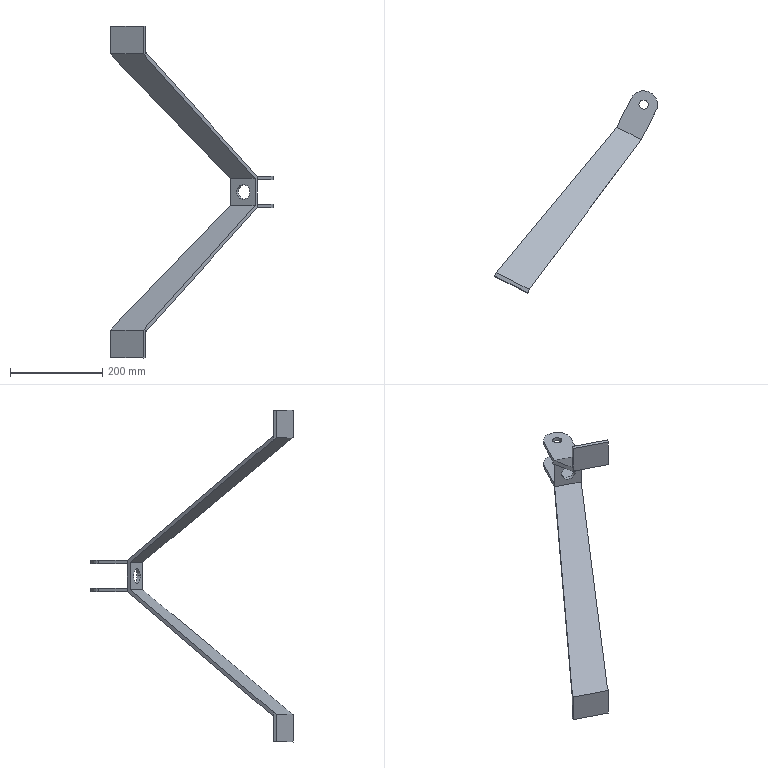Component | SolidWorks | TriangularHanger-1 | 1 solid | 36 faces | box 353.14 x 438.28 x 720 mm | volume 725422 mm3 | plane 26 | cylinder 10 | commonest cylinder face diameters 20 x4 60 x4 32 x2
STEP:
#1=COLOUR_RGB('',0.7922,0.8196,0.9333);
#2=FILL_AREA_STYLE_COLOUR('',#1);
#3=FILL_AREA_STYLE('',(#2));
#4=SURFACE_STYLE_FILL_AREA(#3);
#5=SURFACE_SIDE_STYLE('',(#4));
#6=SURFACE_STYLE_USAGE(.BOTH.,#5);
#7=PRESENTATION_STYLE_ASSIGNMENT((#6));
#8=CARTESIAN_POINT('',(20.97,-29.022,71.377));
#9=VERTEX_POINT('',#8);
#10=CARTESIAN_POINT('',(22.094,-29.591,71.377));
#11=VERTEX_POINT('',#10);
#12=CARTESIAN_POINT('',(21.532,-29.306,71.377));
#13=DIRECTION('',(-0.4521,-0.892,-0.));
#14=DIRECTION('',(0.892,-0.4521,-0.));
#15=AXIS2_PLACEMENT_3D('',#12,#13,#14);
#16=CIRCLE('',#15,0.6299);
#17=EDGE_CURVE('',#9,#11,#16,.T.);
#18=ORIENTED_EDGE('',*,*,#17,.T.);
#19=CARTESIAN_POINT('',(22.236,-29.31,71.377));
#20=VERTEX_POINT('',#19);
#21=CARTESIAN_POINT('',(22.058,-29.661,71.377));
#22=DIRECTION('',(0.4521,0.892,0.));
#23=VECTOR('',#22,39.37);
#24=LINE('',#21,#23);
#25=EDGE_CURVE('',#11,#20,#24,.T.);
#26=ORIENTED_EDGE('',*,*,#25,.T.);
#27=CARTESIAN_POINT('',(21.112,-28.741,71.377));
#28=VERTEX_POINT('',#27);
#29=CARTESIAN_POINT('',(21.674,-29.026,71.377));
#30=DIRECTION('',(0.4521,0.892,0.));
#31=DIRECTION('',(-0.892,0.4521,0.));
#32=AXIS2_PLACEMENT_3D('',#29,#30,#31);
#33=CIRCLE('',#32,0.6299);
#34=EDGE_CURVE('',#20,#28,#33,.T.);
#35=ORIENTED_EDGE('',*,*,#34,.T.);
#36=CARTESIAN_POINT('',(20.934,-29.092,71.377));
#37=DIRECTION('',(0.4521,0.892,0.));
#38=VECTOR('',#37,39.37);
#39=LINE('',#36,#38);
#40=EDGE_CURVE('',#9,#28,#39,.T.);
#41=ORIENTED_EDGE('',*,*,#40,.F.);
#42=EDGE_LOOP('',(#18,#26,#35,#41));
#43=FACE_OUTER_BOUND('',#42,.T.);
#44=CARTESIAN_POINT('',(21.496,-29.377,71.377));
#45=DIRECTION('',(0.4521,0.892,0.));
#46=DIRECTION('',(-0.892,0.4521,0.));
#47=AXIS2_PLACEMENT_3D('',#44,#45,#46);
#48=CYLINDRICAL_SURFACE('',#47,0.6299);
#49=ADVANCED_FACE('',(#43),#48,.F.);
#50=CARTESIAN_POINT('',(22.569,-26.389,70.028));
#51=VERTEX_POINT('',#50);
#52=CARTESIAN_POINT('',(23.271,-26.745,70.028));
#53=VERTEX_POINT('',#52);
#54=CARTESIAN_POINT('',(22.92,-26.567,70.028));
#55=DIRECTION('',(-0.,-0.,1.));
#56=DIRECTION('',(0.892,-0.4521,-0.));
#57=AXIS2_PLACEMENT_3D('',#54,#55,#56);
#58=CIRCLE('',#57,0.3937);
#59=EDGE_CURVE('',#51,#53,#58,.T.);
#60=ORIENTED_EDGE('',*,*,#59,.F.);
#61=CARTESIAN_POINT('',(22.569,-26.389,70.343));
#62=VERTEX_POINT('',#61);
#63=CARTESIAN_POINT('',(22.569,-26.389,68.788));
#64=DIRECTION('',(-0.,-0.,1.));
#65=VECTOR('',#64,39.37);
#66=LINE('',#63,#65);
#67=EDGE_CURVE('',#51,#62,#66,.T.);
#68=ORIENTED_EDGE('',*,*,#67,.T.);
#69=CARTESIAN_POINT('',(23.271,-26.745,70.343));
#70=VERTEX_POINT('',#69);
#71=CARTESIAN_POINT('',(22.92,-26.567,70.343));
#72=DIRECTION('',(0.,0.,-1.));
#73=DIRECTION('',(-0.892,0.4521,0.));
#74=AXIS2_PLACEMENT_3D('',#71,#72,#73);
#75=CIRCLE('',#74,0.3937);
#76=EDGE_CURVE('',#70,#62,#75,.T.);
#77=ORIENTED_EDGE('',*,*,#76,.F.);
#78=CARTESIAN_POINT('',(23.271,-26.745,68.788));
#79=DIRECTION('',(-0.,-0.,1.));
#80=VECTOR('',#79,39.37);
#81=LINE('',#78,#80);
#82=EDGE_CURVE('',#53,#70,#81,.T.);
#83=ORIENTED_EDGE('',*,*,#82,.F.);
#84=EDGE_LOOP('',(#60,#68,#77,#83));
#85=FACE_OUTER_BOUND('',#84,.T.);
#86=CARTESIAN_POINT('',(22.92,-26.567,68.788));
#87=DIRECTION('',(-0.,-0.,1.));
#88=DIRECTION('',(0.892,-0.4521,-0.));
#89=AXIS2_PLACEMENT_3D('',#86,#87,#88);
#90=CYLINDRICAL_SURFACE('',#89,0.3937);
#91=ADVANCED_FACE('',(#85),#90,.F.);
#92=CARTESIAN_POINT('',(22.569,-26.389,72.41));
#93=VERTEX_POINT('',#92);
#94=CARTESIAN_POINT('',(23.271,-26.745,72.41));
#95=VERTEX_POINT('',#94);
#96=CARTESIAN_POINT('',(22.92,-26.567,72.41));
#97=DIRECTION('',(-0.,-0.,1.));
#98=DIRECTION('',(0.892,-0.4521,-0.));
#99=AXIS2_PLACEMENT_3D('',#96,#97,#98);
#100=CIRCLE('',#99,0.3937);
#101=EDGE_CURVE('',#93,#95,#100,.T.);
#102=ORIENTED_EDGE('',*,*,#101,.F.);
#103=CARTESIAN_POINT('',(22.569,-26.389,72.725));
#104=VERTEX_POINT('',#103);
#105=CARTESIAN_POINT('',(22.569,-26.389,68.788));
#106=DIRECTION('',(-0.,-0.,1.));
#107=VECTOR('',#106,39.37);
#108=LINE('',#105,#107);
#109=EDGE_CURVE('',#93,#104,#108,.T.);
#110=ORIENTED_EDGE('',*,*,#109,.T.);
#111=CARTESIAN_POINT('',(23.271,-26.745,72.725));
#112=VERTEX_POINT('',#111);
#113=CARTESIAN_POINT('',(22.92,-26.567,72.725));
#114=DIRECTION('',(-0.,-0.,1.));
#115=DIRECTION('',(0.892,-0.4521,-0.));
#116=AXIS2_PLACEMENT_3D('',#113,#114,#115);
#117=CIRCLE('',#116,0.3937);
#118=EDGE_CURVE('',#104,#112,#117,.T.);
#119=ORIENTED_EDGE('',*,*,#118,.T.);
#120=CARTESIAN_POINT('',(23.271,-26.745,68.788));
#121=DIRECTION('',(-0.,-0.,1.));
#122=VECTOR('',#121,39.37);
#123=LINE('',#120,#122);
#124=EDGE_CURVE('',#95,#112,#123,.T.);
#125=ORIENTED_EDGE('',*,*,#124,.F.);
#126=EDGE_LOOP('',(#102,#110,#119,#125));
#127=FACE_OUTER_BOUND('',#126,.T.);
#128=CARTESIAN_POINT('',(22.92,-26.567,68.788));
#129=DIRECTION('',(-0.,-0.,1.));
#130=DIRECTION('',(0.892,-0.4521,-0.));
#131=AXIS2_PLACEMENT_3D('',#128,#129,#130);
#132=CYLINDRICAL_SURFACE('',#131,0.3937);
#133=ADVANCED_FACE('',(#127),#132,.F.);
#134=CARTESIAN_POINT('',(21.674,-29.026,71.377));
#135=DIRECTION('',(0.4521,0.892,0.));
#136=DIRECTION('',(-0.892,0.4521,0.));
#137=AXIS2_PLACEMENT_3D('',#134,#135,#136);
#138=CIRCLE('',#137,0.6299);
#139=EDGE_CURVE('',#28,#20,#138,.T.);
#140=ORIENTED_EDGE('',*,*,#139,.F.);
#141=ORIENTED_EDGE('',*,*,#34,.F.);
#142=EDGE_LOOP('',(#140,#141));
#143=FACE_BOUND('',#142,.T.);
#144=CARTESIAN_POINT('',(22.728,-29.56,72.41));
#145=VERTEX_POINT('',#144);
#146=CARTESIAN_POINT('',(20.621,-28.492,72.41));
#147=VERTEX_POINT('',#146);
#148=CARTESIAN_POINT('',(22.728,-29.56,72.41));
#149=DIRECTION('',(-0.892,0.4521,0.));
#150=VECTOR('',#149,39.37);
#151=LINE('',#148,#150);
#152=EDGE_CURVE('',#145,#147,#151,.T.);
#153=ORIENTED_EDGE('',*,*,#152,.F.);
#154=CARTESIAN_POINT('',(22.728,-29.56,70.343));
#155=VERTEX_POINT('',#154);
#156=CARTESIAN_POINT('',(22.728,-29.56,70.196));
#157=DIRECTION('',(0.,0.,-1.));
#158=VECTOR('',#157,39.37);
#159=LINE('',#156,#158);
#160=EDGE_CURVE('',#145,#155,#159,.T.);
#161=ORIENTED_EDGE('',*,*,#160,.T.);
#162=CARTESIAN_POINT('',(20.621,-28.492,70.343));
#163=VERTEX_POINT('',#162);
#164=CARTESIAN_POINT('',(22.728,-29.56,70.343));
#165=DIRECTION('',(0.892,-0.4521,-0.));
#166=VECTOR('',#165,39.37);
#167=LINE('',#164,#166);
#168=EDGE_CURVE('',#163,#155,#167,.T.);
#169=ORIENTED_EDGE('',*,*,#168,.F.);
#170=CARTESIAN_POINT('',(20.621,-28.492,52.676));
#171=DIRECTION('',(-0.,-0.,1.));
#172=VECTOR('',#171,39.37);
#173=LINE('',#170,#172);
#174=EDGE_CURVE('',#163,#147,#173,.T.);
#175=ORIENTED_EDGE('',*,*,#174,.T.);
#176=EDGE_LOOP('',(#153,#161,#169,#175));
#177=FACE_OUTER_BOUND('',#176,.T.);
#178=CARTESIAN_POINT('',(17.46,-26.89,70.196));
#179=DIRECTION('',(-0.4521,-0.892,-0.));
#180=DIRECTION('',(0.892,-0.4521,-0.));
#181=AXIS2_PLACEMENT_3D('',#178,#179,#180);
#182=PLANE('',#181);
#183=ADVANCED_FACE('',(#143,#177),#182,.F.);
#184=CARTESIAN_POINT('',(10.341,-40.936,59.398));
#185=VERTEX_POINT('',#184);
#186=CARTESIAN_POINT('',(10.341,-40.936,59.778));
#187=VERTEX_POINT('',#186);
#188=CARTESIAN_POINT('',(10.341,-40.936,71.377));
#189=DIRECTION('',(-0.,-0.,1.));
#190=VECTOR('',#189,39.37);
#191=LINE('',#188,#190);
#192=EDGE_CURVE('',#185,#187,#191,.T.);
#193=ORIENTED_EDGE('',*,*,#192,.F.);
#194=CARTESIAN_POINT('',(10.341,-40.936,57.204));
#195=VERTEX_POINT('',#194);
#196=CARTESIAN_POINT('',(10.341,-40.936,59.566));
#197=DIRECTION('',(0.,0.,-1.));
#198=VECTOR('',#197,39.37);
#199=LINE('',#196,#198);
#200=EDGE_CURVE('',#185,#195,#199,.T.);
#201=ORIENTED_EDGE('',*,*,#200,.T.);
#202=CARTESIAN_POINT('',(10.198,-41.217,57.204));
#203=VERTEX_POINT('',#202);
#204=CARTESIAN_POINT('',(10.198,-41.217,57.204));
#205=DIRECTION('',(0.4521,0.892,0.));
#206=VECTOR('',#205,39.37);
#207=LINE('',#204,#206);
#208=EDGE_CURVE('',#203,#195,#207,.T.);
#209=ORIENTED_EDGE('',*,*,#208,.F.);
#210=CARTESIAN_POINT('',(10.198,-41.217,59.566));
#211=VERTEX_POINT('',#210);
#212=CARTESIAN_POINT('',(10.198,-41.217,59.566));
#213=DIRECTION('',(0.,0.,-1.));
#214=VECTOR('',#213,39.37);
#215=LINE('',#212,#214);
#216=EDGE_CURVE('',#211,#203,#215,.T.);
#217=ORIENTED_EDGE('',*,*,#216,.F.);
#218=CARTESIAN_POINT('',(17.318,-27.171,70.196));
#219=DIRECTION('',(-0.3747,-0.7393,-0.5595));
#220=VECTOR('',#219,39.37);
#221=LINE('',#218,#220);
#222=EDGE_CURVE('',#187,#211,#221,.T.);
#223=ORIENTED_EDGE('',*,*,#222,.F.);
#224=EDGE_LOOP('',(#193,#201,#209,#217,#223));
#225=FACE_OUTER_BOUND('',#224,.T.);
#226=CARTESIAN_POINT('',(10.198,-41.217,71.377));
#227=DIRECTION('',(-0.892,0.4521,0.));
#228=DIRECTION('',(-0.,-0.,1.));
#229=AXIS2_PLACEMENT_3D('',#226,#227,#228);
#230=PLANE('',#229);
#231=ADVANCED_FACE('',(#225),#230,.T.);
#232=CARTESIAN_POINT('',(13.15,-42.36,59.398));
#233=VERTEX_POINT('',#232);
#234=CARTESIAN_POINT('',(10.341,-40.936,59.398));
#235=DIRECTION('',(0.892,-0.4521,-0.));
#236=VECTOR('',#235,39.37);
#237=LINE('',#234,#236);
#238=EDGE_CURVE('',#185,#233,#237,.T.);
#239=ORIENTED_EDGE('',*,*,#238,.T.);
#240=CARTESIAN_POINT('',(13.15,-42.36,57.204));
#241=VERTEX_POINT('',#240);
#242=CARTESIAN_POINT('',(13.15,-42.36,52.676));
#243=DIRECTION('',(-0.,-0.,1.));
#244=VECTOR('',#243,39.37);
#245=LINE('',#242,#244);
#246=EDGE_CURVE('',#241,#233,#245,.T.);
#247=ORIENTED_EDGE('',*,*,#246,.F.);
#248=CARTESIAN_POINT('',(10.341,-40.936,57.204));
#249=DIRECTION('',(0.892,-0.4521,-0.));
#250=VECTOR('',#249,39.37);
#251=LINE('',#248,#250);
#252=EDGE_CURVE('',#195,#241,#251,.T.);
#253=ORIENTED_EDGE('',*,*,#252,.F.);
#254=ORIENTED_EDGE('',*,*,#200,.F.);
#255=EDGE_LOOP('',(#239,#247,#253,#254));
#256=FACE_OUTER_BOUND('',#255,.T.);
#257=CARTESIAN_POINT('',(10.341,-40.936,59.566));
#258=DIRECTION('',(-0.4521,-0.892,-0.));
#259=DIRECTION('',(0.892,-0.4521,-0.));
#260=AXIS2_PLACEMENT_3D('',#257,#258,#259);
#261=PLANE('',#260);
#262=ADVANCED_FACE('',(#256),#261,.F.);
#263=CARTESIAN_POINT('',(13.007,-42.641,57.204));
#264=VERTEX_POINT('',#263);
#265=CARTESIAN_POINT('',(13.007,-42.641,57.204));
#266=DIRECTION('',(0.4521,0.892,0.));
#267=VECTOR('',#266,39.37);
#268=LINE('',#265,#267);
#269=EDGE_CURVE('',#264,#241,#268,.T.);
#270=ORIENTED_EDGE('',*,*,#269,.F.);
#271=CARTESIAN_POINT('',(10.198,-41.217,57.204));
#272=DIRECTION('',(0.892,-0.4521,-0.));
#273=VECTOR('',#272,39.37);
#274=LINE('',#271,#273);
#275=EDGE_CURVE('',#203,#264,#274,.T.);
#276=ORIENTED_EDGE('',*,*,#275,.F.);
#277=ORIENTED_EDGE('',*,*,#208,.T.);
#278=ORIENTED_EDGE('',*,*,#252,.T.);
#279=EDGE_LOOP('',(#270,#276,#277,#278));
#280=FACE_OUTER_BOUND('',#279,.T.);
#281=CARTESIAN_POINT('',(10.198,-41.217,57.204));
#282=DIRECTION('',(0.,0.,-1.));
#283=DIRECTION('',(-0.892,0.4521,0.));
#284=AXIS2_PLACEMENT_3D('',#281,#282,#283);
#285=PLANE('',#284);
#286=ADVANCED_FACE('',(#280),#285,.T.);
#287=CARTESIAN_POINT('',(13.007,-42.641,59.566));
#288=VERTEX_POINT('',#287);
#289=CARTESIAN_POINT('',(13.007,-42.641,52.676));
#290=DIRECTION('',(-0.,-0.,1.));
#291=VECTOR('',#290,39.37);
#292=LINE('',#289,#291);
#293=EDGE_CURVE('',#264,#288,#292,.T.);
#294=ORIENTED_EDGE('',*,*,#293,.T.);
#295=CARTESIAN_POINT('',(10.198,-41.217,59.566));
#296=DIRECTION('',(0.892,-0.4521,-0.));
#297=VECTOR('',#296,39.37);
#298=LINE('',#295,#297);
#299=EDGE_CURVE('',#211,#288,#298,.T.);
#300=ORIENTED_EDGE('',*,*,#299,.F.);
#301=ORIENTED_EDGE('',*,*,#216,.T.);
#302=ORIENTED_EDGE('',*,*,#275,.T.);
#303=EDGE_LOOP('',(#294,#300,#301,#302));
#304=FACE_OUTER_BOUND('',#303,.T.);
#305=CARTESIAN_POINT('',(10.198,-41.217,59.566));
#306=DIRECTION('',(-0.4521,-0.892,-0.));
#307=DIRECTION('',(0.892,-0.4521,-0.));
#308=AXIS2_PLACEMENT_3D('',#305,#306,#307);
#309=PLANE('',#308);
#310=ADVANCED_FACE('',(#304),#309,.T.);
#311=CARTESIAN_POINT('',(13.15,-42.36,59.778));
#312=VERTEX_POINT('',#311);
#313=CARTESIAN_POINT('',(20.127,-28.594,70.196));
#314=DIRECTION('',(-0.3747,-0.7393,-0.5595));
#315=VECTOR('',#314,39.37);
#316=LINE('',#313,#315);
#317=EDGE_CURVE('',#312,#288,#316,.T.);
#318=ORIENTED_EDGE('',*,*,#317,.F.);
#319=CARTESIAN_POINT('',(22.536,-29.816,70.196));
#320=VERTEX_POINT('',#319);
#321=CARTESIAN_POINT('',(22.117,-30.375,69.731));
#322=DIRECTION('',(-0.4989,-0.6668,-0.5537));
#323=VECTOR('',#322,39.37);
#324=LINE('',#321,#323);
#325=EDGE_CURVE('',#320,#312,#324,.T.);
#326=ORIENTED_EDGE('',*,*,#325,.F.);
#327=CARTESIAN_POINT('',(20.415,-28.74,70.196));
#328=VERTEX_POINT('',#327);
#329=CARTESIAN_POINT('',(17.318,-27.171,70.196));
#330=DIRECTION('',(0.892,-0.4521,-0.));
#331=VECTOR('',#330,39.37);
#332=LINE('',#329,#331);
#333=EDGE_CURVE('',#328,#320,#332,.T.);
#334=ORIENTED_EDGE('',*,*,#333,.F.);
#335=CARTESIAN_POINT('',(20.077,-29.15,69.846));
#336=DIRECTION('',(0.5319,0.6439,0.55));
#337=VECTOR('',#336,39.37);
#338=LINE('',#335,#337);
#339=EDGE_CURVE('',#187,#328,#338,.T.);
#340=ORIENTED_EDGE('',*,*,#339,.F.);
#341=ORIENTED_EDGE('',*,*,#222,.T.);
#342=ORIENTED_EDGE('',*,*,#299,.T.);
#343=EDGE_LOOP('',(#318,#326,#334,#340,#341,#342));
#344=FACE_OUTER_BOUND('',#343,.T.);
#345=CARTESIAN_POINT('',(17.318,-27.171,70.196));
#346=DIRECTION('',(-0.2529,-0.499,0.8288));
#347=DIRECTION('',(0.3747,0.7393,0.5595));
#348=AXIS2_PLACEMENT_3D('',#345,#346,#347);
#349=PLANE('',#348);
#350=ADVANCED_FACE('',(#344),#349,.T.);
#351=ORIENTED_EDGE('',*,*,#17,.F.);
#352=CARTESIAN_POINT('',(21.532,-29.306,71.377));
#353=DIRECTION('',(-0.4521,-0.892,-0.));
#354=DIRECTION('',(0.892,-0.4521,-0.));
#355=AXIS2_PLACEMENT_3D('',#352,#353,#354);
#356=CIRCLE('',#355,0.6299);
#357=EDGE_CURVE('',#11,#9,#356,.T.);
#358=ORIENTED_EDGE('',*,*,#357,.F.);
#359=EDGE_LOOP('',(#351,#358));
#360=FACE_BOUND('',#359,.T.);
#361=CARTESIAN_POINT('',(22.536,-29.816,72.558));
#362=VERTEX_POINT('',#361);
#363=CARTESIAN_POINT('',(22.536,-29.816,70.196));
#364=DIRECTION('',(0.,0.,-1.));
#365=VECTOR('',#364,39.37);
#366=LINE('',#363,#365);
#367=EDGE_CURVE('',#362,#320,#366,.T.);
#368=ORIENTED_EDGE('',*,*,#367,.F.);
#369=CARTESIAN_POINT('',(20.415,-28.74,72.558));
#370=VERTEX_POINT('',#369);
#371=CARTESIAN_POINT('',(17.318,-27.171,72.558));
#372=DIRECTION('',(0.892,-0.4521,-0.));
#373=VECTOR('',#372,39.37);
#374=LINE('',#371,#373);
#375=EDGE_CURVE('',#370,#362,#374,.T.);
#376=ORIENTED_EDGE('',*,*,#375,.F.);
#377=CARTESIAN_POINT('',(20.415,-28.74,70.196));
#378=DIRECTION('',(-0.,-0.,1.));
#379=VECTOR('',#378,39.37);
#380=LINE('',#377,#379);
#381=EDGE_CURVE('',#328,#370,#380,.T.);
#382=ORIENTED_EDGE('',*,*,#381,.F.);
#383=ORIENTED_EDGE('',*,*,#333,.T.);
#384=EDGE_LOOP('',(#368,#376,#382,#383));
#385=FACE_OUTER_BOUND('',#384,.T.);
#386=CARTESIAN_POINT('',(17.318,-27.171,70.196));
#387=DIRECTION('',(-0.4521,-0.892,-0.));
#388=DIRECTION('',(0.892,-0.4521,-0.));
#389=AXIS2_PLACEMENT_3D('',#386,#387,#388);
#390=PLANE('',#389);
#391=ADVANCED_FACE('',(#360,#385),#390,.T.);
#392=CARTESIAN_POINT('',(13.007,-42.641,83.188));
#393=VERTEX_POINT('',#392);
#394=CARTESIAN_POINT('',(13.15,-42.36,82.975));
#395=VERTEX_POINT('',#394);
#396=CARTESIAN_POINT('',(20.127,-28.594,72.558));
#397=DIRECTION('',(0.3747,0.7393,-0.5595));
#398=VECTOR('',#397,39.37);
#399=LINE('',#396,#398);
#400=EDGE_CURVE('',#393,#395,#399,.T.);
#401=ORIENTED_EDGE('',*,*,#400,.F.);
#402=CARTESIAN_POINT('',(10.198,-41.217,83.188));
#403=VERTEX_POINT('',#402);
#404=CARTESIAN_POINT('',(10.198,-41.217,83.188));
#405=DIRECTION('',(0.892,-0.4521,-0.));
#406=VECTOR('',#405,39.37);
#407=LINE('',#404,#406);
#408=EDGE_CURVE('',#403,#393,#407,.T.);
#409=ORIENTED_EDGE('',*,*,#408,.F.);
#410=CARTESIAN_POINT('',(10.341,-40.936,82.975));
#411=VERTEX_POINT('',#410);
#412=CARTESIAN_POINT('',(17.318,-27.171,72.558));
#413=DIRECTION('',(0.3747,0.7393,-0.5595));
#414=VECTOR('',#413,39.37);
#415=LINE('',#412,#414);
#416=EDGE_CURVE('',#403,#411,#415,.T.);
#417=ORIENTED_EDGE('',*,*,#416,.T.);
#418=CARTESIAN_POINT('',(20.077,-29.15,72.908));
#419=DIRECTION('',(-0.5319,-0.6439,0.55));
#420=VECTOR('',#419,39.37);
#421=LINE('',#418,#420);
#422=EDGE_CURVE('',#370,#411,#421,.T.);
#423=ORIENTED_EDGE('',*,*,#422,.F.);
#424=ORIENTED_EDGE('',*,*,#375,.T.);
#425=CARTESIAN_POINT('',(22.117,-30.375,73.023));
#426=DIRECTION('',(0.4989,0.6668,-0.5537));
#427=VECTOR('',#426,39.37);
#428=LINE('',#425,#427);
#429=EDGE_CURVE('',#395,#362,#428,.T.);
#430=ORIENTED_EDGE('',*,*,#429,.F.);
#431=EDGE_LOOP('',(#401,#409,#417,#423,#424,#430));
#432=FACE_OUTER_BOUND('',#431,.T.);
#433=CARTESIAN_POINT('',(17.318,-27.171,72.558));
#434=DIRECTION('',(-0.2529,-0.499,-0.8288));
#435=DIRECTION('',(-0.3747,-0.7393,0.5595));
#436=AXIS2_PLACEMENT_3D('',#433,#434,#435);
#437=PLANE('',#436);
#438=ADVANCED_FACE('',(#432),#437,.T.);
#439=CARTESIAN_POINT('',(13.007,-42.641,85.55));
#440=VERTEX_POINT('',#439);
#441=CARTESIAN_POINT('',(13.007,-42.641,52.676));
#442=DIRECTION('',(-0.,-0.,1.));
#443=VECTOR('',#442,39.37);
#444=LINE('',#441,#443);
#445=EDGE_CURVE('',#393,#440,#444,.T.);
#446=ORIENTED_EDGE('',*,*,#445,.T.);
#447=CARTESIAN_POINT('',(10.198,-41.217,85.55));
#448=VERTEX_POINT('',#447);
#449=CARTESIAN_POINT('',(10.198,-41.217,85.55));
#450=DIRECTION('',(0.892,-0.4521,-0.));
#451=VECTOR('',#450,39.37);
#452=LINE('',#449,#451);
#453=EDGE_CURVE('',#448,#440,#452,.T.);
#454=ORIENTED_EDGE('',*,*,#453,.F.);
#455=CARTESIAN_POINT('',(10.198,-41.217,83.188));
#456=DIRECTION('',(0.,0.,-1.));
#457=VECTOR('',#456,39.37);
#458=LINE('',#455,#457);
#459=EDGE_CURVE('',#448,#403,#458,.T.);
#460=ORIENTED_EDGE('',*,*,#459,.T.);
#461=ORIENTED_EDGE('',*,*,#408,.T.);
#462=EDGE_LOOP('',(#446,#454,#460,#461));
#463=FACE_OUTER_BOUND('',#462,.T.);
#464=CARTESIAN_POINT('',(10.198,-41.217,83.188));
#465=DIRECTION('',(-0.4521,-0.892,-0.));
#466=DIRECTION('',(0.892,-0.4521,-0.));
#467=AXIS2_PLACEMENT_3D('',#464,#465,#466);
#468=PLANE('',#467);
#469=ADVANCED_FACE('',(#463),#468,.T.);
#470=CARTESIAN_POINT('',(13.15,-42.36,85.55));
#471=VERTEX_POINT('',#470);
#472=CARTESIAN_POINT('',(13.15,-42.36,85.55));
#473=DIRECTION('',(-0.4521,-0.892,-0.));
#474=VECTOR('',#473,39.37);
#475=LINE('',#472,#474);
#476=EDGE_CURVE('',#471,#440,#475,.T.);
#477=ORIENTED_EDGE('',*,*,#476,.F.);
#478=CARTESIAN_POINT('',(10.341,-40.936,85.55));
#479=VERTEX_POINT('',#478);
#480=CARTESIAN_POINT('',(10.341,-40.936,85.55));
#481=DIRECTION('',(0.892,-0.4521,-0.));
#482=VECTOR('',#481,39.37);
#483=LINE('',#480,#482);
#484=EDGE_CURVE('',#479,#471,#483,.T.);
#485=ORIENTED_EDGE('',*,*,#484,.F.);
#486=CARTESIAN_POINT('',(10.341,-40.936,85.55));
#487=DIRECTION('',(-0.4521,-0.892,-0.));
#488=VECTOR('',#487,39.37);
#489=LINE('',#486,#488);
#490=EDGE_CURVE('',#479,#448,#489,.T.);
#491=ORIENTED_EDGE('',*,*,#490,.T.);
#492=ORIENTED_EDGE('',*,*,#453,.T.);
#493=EDGE_LOOP('',(#477,#485,#491,#492));
#494=FACE_OUTER_BOUND('',#493,.T.);
#495=CARTESIAN_POINT('',(10.341,-40.936,85.55));
#496=DIRECTION('',(-0.,-0.,1.));
#497=DIRECTION('',(0.892,-0.4521,-0.));
#498=AXIS2_PLACEMENT_3D('',#495,#496,#497);
#499=PLANE('',#498);
#500=ADVANCED_FACE('',(#494),#499,.T.);
#501=ORIENTED_EDGE('',*,*,#484,.T.);
#502=CARTESIAN_POINT('',(13.15,-42.36,83.355));
#503=VERTEX_POINT('',#502);
#504=CARTESIAN_POINT('',(13.15,-42.36,52.676));
#505=DIRECTION('',(-0.,-0.,1.));
#506=VECTOR('',#505,39.37);
#507=LINE('',#504,#506);
#508=EDGE_CURVE('',#503,#471,#507,.T.);
#509=ORIENTED_EDGE('',*,*,#508,.F.);
#510=CARTESIAN_POINT('',(10.341,-40.936,83.355));
#511=VERTEX_POINT('',#510);
#512=CARTESIAN_POINT('',(10.341,-40.936,83.355));
#513=DIRECTION('',(0.892,-0.4521,-0.));
#514=VECTOR('',#513,39.37);
#515=LINE('',#512,#514);
#516=EDGE_CURVE('',#511,#503,#515,.T.);
#517=ORIENTED_EDGE('',*,*,#516,.F.);
#518=CARTESIAN_POINT('',(10.341,-40.936,83.188));
#519=DIRECTION('',(0.,0.,-1.));
#520=VECTOR('',#519,39.37);
#521=LINE('',#518,#520);
#522=EDGE_CURVE('',#479,#511,#521,.T.);
#523=ORIENTED_EDGE('',*,*,#522,.F.);
#524=EDGE_LOOP('',(#501,#509,#517,#523));
#525=FACE_OUTER_BOUND('',#524,.T.);
#526=CARTESIAN_POINT('',(10.341,-40.936,83.188));
#527=DIRECTION('',(-0.4521,-0.892,-0.));
#528=DIRECTION('',(0.892,-0.4521,-0.));
#529=AXIS2_PLACEMENT_3D('',#526,#527,#528);
#530=PLANE('',#529);
#531=ADVANCED_FACE('',(#525),#530,.F.);
#532=ORIENTED_EDGE('',*,*,#516,.T.);
#533=CARTESIAN_POINT('',(22.728,-29.56,72.725));
#534=VERTEX_POINT('',#533);
#535=CARTESIAN_POINT('',(22.222,-30.235,73.286));
#536=DIRECTION('',(0.4989,0.6668,-0.5537));
#537=VECTOR('',#536,39.37);
#538=LINE('',#535,#537);
#539=EDGE_CURVE('',#503,#534,#538,.T.);
#540=ORIENTED_EDGE('',*,*,#539,.T.);
#541=CARTESIAN_POINT('',(20.621,-28.492,72.725));
#542=VERTEX_POINT('',#541);
#543=CARTESIAN_POINT('',(17.46,-26.89,72.725));
#544=DIRECTION('',(0.892,-0.4521,-0.));
#545=VECTOR('',#544,39.37);
#546=LINE('',#543,#545);
#547=EDGE_CURVE('',#542,#534,#546,.T.);
#548=ORIENTED_EDGE('',*,*,#547,.F.);
#549=CARTESIAN_POINT('',(20.188,-29.016,73.173));
#550=DIRECTION('',(-0.5319,-0.6439,0.55));
#551=VECTOR('',#550,39.37);
#552=LINE('',#549,#551);
#553=EDGE_CURVE('',#542,#511,#552,.T.);
#554=ORIENTED_EDGE('',*,*,#553,.T.);
#555=EDGE_LOOP('',(#532,#540,#548,#554));
#556=FACE_OUTER_BOUND('',#555,.T.);
#557=CARTESIAN_POINT('',(17.398,-27.013,72.819));
#558=DIRECTION('',(-0.2529,-0.499,-0.8288));
#559=DIRECTION('',(-0.3747,-0.7393,0.5595));
#560=AXIS2_PLACEMENT_3D('',#557,#558,#559);
#561=PLANE('',#560);
#562=ADVANCED_FACE('',(#556),#561,.F.);
#563=CARTESIAN_POINT('',(20.621,-28.492,70.028));
#564=VERTEX_POINT('',#563);
#565=CARTESIAN_POINT('',(22.728,-29.56,70.028));
#566=VERTEX_POINT('',#565);
#567=CARTESIAN_POINT('',(17.46,-26.89,70.028));
#568=DIRECTION('',(0.892,-0.4521,-0.));
#569=VECTOR('',#568,39.37);
#570=LINE('',#567,#569);
#571=EDGE_CURVE('',#564,#566,#570,.T.);
#572=ORIENTED_EDGE('',*,*,#571,.T.);
#573=CARTESIAN_POINT('',(22.222,-30.235,69.467));
#574=DIRECTION('',(-0.4989,-0.6668,-0.5537));
#575=VECTOR('',#574,39.37);
#576=LINE('',#573,#575);
#577=EDGE_CURVE('',#566,#233,#576,.T.);
#578=ORIENTED_EDGE('',*,*,#577,.T.);
#579=ORIENTED_EDGE('',*,*,#238,.F.);
#580=CARTESIAN_POINT('',(20.188,-29.016,69.581));
#581=DIRECTION('',(0.5319,0.6439,0.55));
#582=VECTOR('',#581,39.37);
#583=LINE('',#580,#582);
#584=EDGE_CURVE('',#185,#564,#583,.T.);
#585=ORIENTED_EDGE('',*,*,#584,.T.);
#586=EDGE_LOOP('',(#572,#578,#579,#585));
#587=FACE_OUTER_BOUND('',#586,.T.);
#588=CARTESIAN_POINT('',(17.398,-27.013,69.935));
#589=DIRECTION('',(-0.2529,-0.499,0.8288));
#590=DIRECTION('',(0.3747,0.7393,0.5595));
#591=AXIS2_PLACEMENT_3D('',#588,#589,#590);
#592=PLANE('',#591);
#593=ADVANCED_FACE('',(#587),#592,.F.);
#594=CARTESIAN_POINT('',(10.341,-40.936,71.377));
#595=DIRECTION('',(-0.,-0.,1.));
#596=VECTOR('',#595,39.37);
#597=LINE('',#594,#596);
#598=EDGE_CURVE('',#411,#511,#597,.T.);
#599=ORIENTED_EDGE('',*,*,#598,.F.);
#600=ORIENTED_EDGE('',*,*,#416,.F.);
#601=ORIENTED_EDGE('',*,*,#459,.F.);
#602=ORIENTED_EDGE('',*,*,#490,.F.);
#603=ORIENTED_EDGE('',*,*,#522,.T.);
#604=EDGE_LOOP('',(#599,#600,#601,#602,#603));
#605=FACE_OUTER_BOUND('',#604,.T.);
#606=CARTESIAN_POINT('',(10.198,-41.217,71.377));
#607=DIRECTION('',(-0.892,0.4521,0.));
#608=DIRECTION('',(-0.,-0.,1.));
#609=AXIS2_PLACEMENT_3D('',#606,#607,#608);
#610=PLANE('',#609);
#611=ADVANCED_FACE('',(#605),#610,.T.);
#612=ORIENTED_EDGE('',*,*,#339,.T.);
#613=ORIENTED_EDGE('',*,*,#381,.T.);
#614=ORIENTED_EDGE('',*,*,#422,.T.);
#615=ORIENTED_EDGE('',*,*,#598,.T.);
#616=ORIENTED_EDGE('',*,*,#553,.F.);
#617=CARTESIAN_POINT('',(20.621,-28.492,72.725));
#618=DIRECTION('',(-0.,-0.,1.));
#619=VECTOR('',#618,39.37);
#620=LINE('',#617,#619);
#621=EDGE_CURVE('',#147,#542,#620,.T.);
#622=ORIENTED_EDGE('',*,*,#621,.F.);
#623=ORIENTED_EDGE('',*,*,#174,.F.);
#624=CARTESIAN_POINT('',(20.621,-28.492,52.676));
#625=DIRECTION('',(-0.,-0.,1.));
#626=VECTOR('',#625,39.37);
#627=LINE('',#624,#626);
#628=EDGE_CURVE('',#564,#163,#627,.T.);
#629=ORIENTED_EDGE('',*,*,#628,.F.);
#630=ORIENTED_EDGE('',*,*,#584,.F.);
#631=ORIENTED_EDGE('',*,*,#192,.T.);
#632=EDGE_LOOP('',(#612,#613,#614,#615,#616,#622,#623,#629,#630,#631));
#633=FACE_OUTER_BOUND('',#632,.T.);
#634=CARTESIAN_POINT('',(20.621,-28.492,52.676));
#635=DIRECTION('',(0.771,-0.6369,-0.));
#636=DIRECTION('',(0.6369,0.771,0.));
#637=AXIS2_PLACEMENT_3D('',#634,#635,#636);
#638=PLANE('',#637);
#639=ADVANCED_FACE('',(#633),#638,.F.);
#640=ORIENTED_EDGE('',*,*,#269,.T.);
#641=ORIENTED_EDGE('',*,*,#246,.T.);
#642=CARTESIAN_POINT('',(13.15,-42.36,52.676));
#643=DIRECTION('',(-0.,-0.,1.));
#644=VECTOR('',#643,39.37);
#645=LINE('',#642,#644);
#646=EDGE_CURVE('',#233,#312,#645,.T.);
#647=ORIENTED_EDGE('',*,*,#646,.T.);
#648=ORIENTED_EDGE('',*,*,#317,.T.);
#649=ORIENTED_EDGE('',*,*,#293,.F.);
#650=EDGE_LOOP('',(#640,#641,#647,#648,#649));
#651=FACE_OUTER_BOUND('',#650,.T.);
#652=CARTESIAN_POINT('',(13.15,-42.36,52.676));
#653=DIRECTION('',(-0.892,0.4521,0.));
#654=DIRECTION('',(-0.,-0.,1.));
#655=AXIS2_PLACEMENT_3D('',#652,#653,#654);
#656=PLANE('',#655);
#657=ADVANCED_FACE('',(#651),#656,.F.);
#658=ORIENTED_EDGE('',*,*,#325,.T.);
#659=ORIENTED_EDGE('',*,*,#646,.F.);
#660=ORIENTED_EDGE('',*,*,#577,.F.);
#661=CARTESIAN_POINT('',(22.728,-29.56,70.028));
#662=DIRECTION('',(0.,0.,-1.));
#663=VECTOR('',#662,39.37);
#664=LINE('',#661,#663);
#665=EDGE_CURVE('',#155,#566,#664,.T.);
#666=ORIENTED_EDGE('',*,*,#665,.F.);
#667=ORIENTED_EDGE('',*,*,#160,.F.);
#668=CARTESIAN_POINT('',(22.728,-29.56,70.196));
#669=DIRECTION('',(0.,0.,-1.));
#670=VECTOR('',#669,39.37);
#671=LINE('',#668,#670);
#672=EDGE_CURVE('',#534,#145,#671,.T.);
#673=ORIENTED_EDGE('',*,*,#672,.F.);
#674=ORIENTED_EDGE('',*,*,#539,.F.);
#675=CARTESIAN_POINT('',(13.15,-42.36,52.676));
#676=DIRECTION('',(-0.,-0.,1.));
#677=VECTOR('',#676,39.37);
#678=LINE('',#675,#677);
#679=EDGE_CURVE('',#395,#503,#678,.T.);
#680=ORIENTED_EDGE('',*,*,#679,.F.);
#681=ORIENTED_EDGE('',*,*,#429,.T.);
#682=ORIENTED_EDGE('',*,*,#367,.T.);
#683=EDGE_LOOP('',(#658,#659,#660,#666,#667,#673,#674,#680,#681,#682));
#684=FACE_OUTER_BOUND('',#683,.T.);
#685=CARTESIAN_POINT('',(22.728,-29.56,52.676));
#686=DIRECTION('',(-0.8007,0.5991,0.));
#687=DIRECTION('',(-0.5991,-0.8007,-0.));
#688=AXIS2_PLACEMENT_3D('',#685,#686,#687);
#689=PLANE('',#688);
#690=ADVANCED_FACE('',(#684),#689,.F.);
#691=ORIENTED_EDGE('',*,*,#400,.T.);
#692=ORIENTED_EDGE('',*,*,#679,.T.);
#693=ORIENTED_EDGE('',*,*,#508,.T.);
#694=ORIENTED_EDGE('',*,*,#476,.T.);
#695=ORIENTED_EDGE('',*,*,#445,.F.);
#696=EDGE_LOOP('',(#691,#692,#693,#694,#695));
#697=FACE_OUTER_BOUND('',#696,.T.);
#698=CARTESIAN_POINT('',(13.15,-42.36,52.676));
#699=DIRECTION('',(-0.892,0.4521,0.));
#700=DIRECTION('',(-0.,-0.,1.));
#701=AXIS2_PLACEMENT_3D('',#698,#699,#700);
#702=PLANE('',#701);
#703=ADVANCED_FACE('',(#697),#702,.F.);
#704=CARTESIAN_POINT('',(22.92,-26.567,70.028));
#705=DIRECTION('',(-0.,-0.,1.));
#706=DIRECTION('',(0.892,-0.4521,-0.));
#707=AXIS2_PLACEMENT_3D('',#704,#705,#706);
#708=CIRCLE('',#707,0.3937);
#709=EDGE_CURVE('',#53,#51,#708,.T.);
#710=ORIENTED_EDGE('',*,*,#709,.T.);
#711=ORIENTED_EDGE('',*,*,#59,.T.);
#712=EDGE_LOOP('',(#710,#711));
#713=FACE_BOUND('',#712,.T.);
#714=CARTESIAN_POINT('',(21.867,-26.033,70.028));
#715=VERTEX_POINT('',#714);
#716=CARTESIAN_POINT('',(22.401,-24.98,70.028));
#717=DIRECTION('',(-0.4521,-0.892,-0.));
#718=VECTOR('',#717,39.37);
#719=LINE('',#716,#718);
#720=EDGE_CURVE('',#715,#564,#719,.T.);
#721=ORIENTED_EDGE('',*,*,#720,.F.);
#722=CARTESIAN_POINT('',(23.454,-25.514,70.028));
#723=VERTEX_POINT('',#722);
#724=CARTESIAN_POINT('',(22.92,-26.567,70.028));
#725=DIRECTION('',(0.,0.,-1.));
#726=DIRECTION('',(0.892,-0.4521,-0.));
#727=AXIS2_PLACEMENT_3D('',#724,#725,#726);
#728=CIRCLE('',#727,1.181);
#729=EDGE_CURVE('',#715,#723,#728,.T.);
#730=ORIENTED_EDGE('',*,*,#729,.T.);
#731=CARTESIAN_POINT('',(23.974,-27.101,70.028));
#732=VERTEX_POINT('',#731);
#733=CARTESIAN_POINT('',(22.92,-26.567,70.028));
#734=DIRECTION('',(0.,0.,-1.));
#735=DIRECTION('',(0.892,-0.4521,-0.));
#736=AXIS2_PLACEMENT_3D('',#733,#734,#735);
#737=CIRCLE('',#736,1.181);
#738=EDGE_CURVE('',#723,#732,#737,.T.);
#739=ORIENTED_EDGE('',*,*,#738,.T.);
#740=CARTESIAN_POINT('',(24.508,-26.048,70.028));
#741=DIRECTION('',(-0.4521,-0.892,-0.));
#742=VECTOR('',#741,39.37);
#743=LINE('',#740,#742);
#744=EDGE_CURVE('',#732,#566,#743,.T.);
#745=ORIENTED_EDGE('',*,*,#744,.T.);
#746=ORIENTED_EDGE('',*,*,#571,.F.);
#747=EDGE_LOOP('',(#721,#730,#739,#745,#746));
#748=FACE_OUTER_BOUND('',#747,.T.);
#749=CARTESIAN_POINT('',(24.508,-26.048,70.028));
#750=DIRECTION('',(-0.,-0.,1.));
#751=DIRECTION('',(0.892,-0.4521,-0.));
#752=AXIS2_PLACEMENT_3D('',#749,#750,#751);
#753=PLANE('',#752);
#754=ADVANCED_FACE('',(#713,#748),#753,.F.);
#755=CARTESIAN_POINT('',(21.867,-26.033,70.343));
#756=VERTEX_POINT('',#755);
#757=CARTESIAN_POINT('',(22.401,-24.98,70.343));
#758=DIRECTION('',(-0.4521,-0.892,-0.));
#759=VECTOR('',#758,39.37);
#760=LINE('',#757,#759);
#761=EDGE_CURVE('',#756,#163,#760,.T.);
#762=ORIENTED_EDGE('',*,*,#761,.F.);
#763=CARTESIAN_POINT('',(21.867,-26.033,70.028));
#764=DIRECTION('',(0.,0.,-1.));
#765=VECTOR('',#764,39.37);
#766=LINE('',#763,#765);
#767=EDGE_CURVE('',#756,#715,#766,.T.);
#768=ORIENTED_EDGE('',*,*,#767,.T.);
#769=ORIENTED_EDGE('',*,*,#720,.T.);
#770=ORIENTED_EDGE('',*,*,#628,.T.);
#771=EDGE_LOOP('',(#762,#768,#769,#770));
#772=FACE_OUTER_BOUND('',#771,.T.);
#773=CARTESIAN_POINT('',(22.401,-24.98,70.028));
#774=DIRECTION('',(0.892,-0.4521,-0.));
#775=DIRECTION('',(0.,0.,-1.));
#776=AXIS2_PLACEMENT_3D('',#773,#774,#775);
#777=PLANE('',#776);
#778=ADVANCED_FACE('',(#772),#777,.F.);
#779=ORIENTED_EDGE('',*,*,#76,.T.);
#780=CARTESIAN_POINT('',(22.92,-26.567,70.343));
#781=DIRECTION('',(0.,0.,-1.));
#782=DIRECTION('',(-0.892,0.4521,0.));
#783=AXIS2_PLACEMENT_3D('',#780,#781,#782);
#784=CIRCLE('',#783,0.3937);
#785=EDGE_CURVE('',#62,#70,#784,.T.);
#786=ORIENTED_EDGE('',*,*,#785,.T.);
#787=EDGE_LOOP('',(#779,#786));
#788=FACE_BOUND('',#787,.T.);
#789=CARTESIAN_POINT('',(23.974,-27.101,70.343));
#790=VERTEX_POINT('',#789);
#791=CARTESIAN_POINT('',(23.454,-25.514,70.343));
#792=VERTEX_POINT('',#791);
#793=CARTESIAN_POINT('',(22.92,-26.567,70.343));
#794=DIRECTION('',(-0.,-0.,1.));
#795=DIRECTION('',(-0.892,0.4521,0.));
#796=AXIS2_PLACEMENT_3D('',#793,#794,#795);
#797=CIRCLE('',#796,1.181);
#798=EDGE_CURVE('',#790,#792,#797,.T.);
#799=ORIENTED_EDGE('',*,*,#798,.T.);
#800=CARTESIAN_POINT('',(22.92,-26.567,70.343));
#801=DIRECTION('',(-0.,-0.,1.));
#802=DIRECTION('',(-0.892,0.4521,0.));
#803=AXIS2_PLACEMENT_3D('',#800,#801,#802);
#804=CIRCLE('',#803,1.181);
#805=EDGE_CURVE('',#792,#756,#804,.T.);
#806=ORIENTED_EDGE('',*,*,#805,.T.);
#807=ORIENTED_EDGE('',*,*,#761,.T.);
#808=ORIENTED_EDGE('',*,*,#168,.T.);
#809=CARTESIAN_POINT('',(24.508,-26.048,70.343));
#810=DIRECTION('',(-0.4521,-0.892,-0.));
#811=VECTOR('',#810,39.37);
#812=LINE('',#809,#811);
#813=EDGE_CURVE('',#790,#155,#812,.T.);
#814=ORIENTED_EDGE('',*,*,#813,.F.);
#815=EDGE_LOOP('',(#799,#806,#807,#808,#814));
#816=FACE_OUTER_BOUND('',#815,.T.);
#817=CARTESIAN_POINT('',(24.508,-26.048,70.343));
#818=DIRECTION('',(0.,0.,-1.));
#819=DIRECTION('',(-0.892,0.4521,0.));
#820=AXIS2_PLACEMENT_3D('',#817,#818,#819);
#821=PLANE('',#820);
#822=ADVANCED_FACE('',(#788,#816),#821,.F.);
#823=ORIENTED_EDGE('',*,*,#744,.F.);
#824=CARTESIAN_POINT('',(23.974,-27.101,70.343));
#825=DIRECTION('',(-0.,-0.,1.));
#826=VECTOR('',#825,39.37);
#827=LINE('',#824,#826);
#828=EDGE_CURVE('',#732,#790,#827,.T.);
#829=ORIENTED_EDGE('',*,*,#828,.T.);
#830=ORIENTED_EDGE('',*,*,#813,.T.);
#831=ORIENTED_EDGE('',*,*,#665,.T.);
#832=EDGE_LOOP('',(#823,#829,#830,#831));
#833=FACE_OUTER_BOUND('',#832,.T.);
#834=CARTESIAN_POINT('',(24.508,-26.048,70.028));
#835=DIRECTION('',(-0.892,0.4521,0.));
#836=DIRECTION('',(-0.,-0.,1.));
#837=AXIS2_PLACEMENT_3D('',#834,#835,#836);
#838=PLANE('',#837);
#839=ADVANCED_FACE('',(#833),#838,.F.);
#840=CARTESIAN_POINT('',(22.92,-26.567,72.725));
#841=DIRECTION('',(-0.,-0.,1.));
#842=DIRECTION('',(0.892,-0.4521,-0.));
#843=AXIS2_PLACEMENT_3D('',#840,#841,#842);
#844=CIRCLE('',#843,0.3937);
#845=EDGE_CURVE('',#112,#104,#844,.T.);
#846=ORIENTED_EDGE('',*,*,#845,.F.);
#847=ORIENTED_EDGE('',*,*,#118,.F.);
#848=EDGE_LOOP('',(#846,#847));
#849=FACE_BOUND('',#848,.T.);
#850=CARTESIAN_POINT('',(23.974,-27.101,72.725));
#851=VERTEX_POINT('',#850);
#852=CARTESIAN_POINT('',(23.454,-25.514,72.725));
#853=VERTEX_POINT('',#852);
#854=CARTESIAN_POINT('',(22.92,-26.567,72.725));
#855=DIRECTION('',(-0.,-0.,1.));
#856=DIRECTION('',(-0.892,0.4521,0.));
#857=AXIS2_PLACEMENT_3D('',#854,#855,#856);
#858=CIRCLE('',#857,1.181);
#859=EDGE_CURVE('',#851,#853,#858,.T.);
#860=ORIENTED_EDGE('',*,*,#859,.T.);
#861=CARTESIAN_POINT('',(21.867,-26.033,72.725));
#862=VERTEX_POINT('',#861);
#863=CARTESIAN_POINT('',(22.92,-26.567,72.725));
#864=DIRECTION('',(-0.,-0.,1.));
#865=DIRECTION('',(-0.892,0.4521,0.));
#866=AXIS2_PLACEMENT_3D('',#863,#864,#865);
#867=CIRCLE('',#866,1.181);
#868=EDGE_CURVE('',#853,#862,#867,.T.);
#869=ORIENTED_EDGE('',*,*,#868,.T.);
#870=CARTESIAN_POINT('',(22.401,-24.98,72.725));
#871=DIRECTION('',(-0.4521,-0.892,-0.));
#872=VECTOR('',#871,39.37);
#873=LINE('',#870,#872);
#874=EDGE_CURVE('',#862,#542,#873,.T.);
#875=ORIENTED_EDGE('',*,*,#874,.T.);
#876=ORIENTED_EDGE('',*,*,#547,.T.);
#877=CARTESIAN_POINT('',(24.508,-26.048,72.725));
#878=DIRECTION('',(-0.4521,-0.892,-0.));
#879=VECTOR('',#878,39.37);
#880=LINE('',#877,#879);
#881=EDGE_CURVE('',#851,#534,#880,.T.);
#882=ORIENTED_EDGE('',*,*,#881,.F.);
#883=EDGE_LOOP('',(#860,#869,#875,#876,#882));
#884=FACE_OUTER_BOUND('',#883,.T.);
#885=CARTESIAN_POINT('',(24.508,-26.048,72.725));
#886=DIRECTION('',(0.,0.,-1.));
#887=DIRECTION('',(-0.892,0.4521,0.));
#888=AXIS2_PLACEMENT_3D('',#885,#886,#887);
#889=PLANE('',#888);
#890=ADVANCED_FACE('',(#849,#884),#889,.F.);
#891=CARTESIAN_POINT('',(23.974,-27.101,72.41));
#892=VERTEX_POINT('',#891);
#893=CARTESIAN_POINT('',(24.508,-26.048,72.41));
#894=DIRECTION('',(-0.4521,-0.892,-0.));
#895=VECTOR('',#894,39.37);
#896=LINE('',#893,#895);
#897=EDGE_CURVE('',#892,#145,#896,.T.);
#898=ORIENTED_EDGE('',*,*,#897,.F.);
#899=CARTESIAN_POINT('',(23.974,-27.101,72.725));
#900=DIRECTION('',(-0.,-0.,1.));
#901=VECTOR('',#900,39.37);
#902=LINE('',#899,#901);
#903=EDGE_CURVE('',#892,#851,#902,.T.);
#904=ORIENTED_EDGE('',*,*,#903,.T.);
#905=ORIENTED_EDGE('',*,*,#881,.T.);
#906=ORIENTED_EDGE('',*,*,#672,.T.);
#907=EDGE_LOOP('',(#898,#904,#905,#906));
#908=FACE_OUTER_BOUND('',#907,.T.);
#909=CARTESIAN_POINT('',(24.508,-26.048,72.725));
#910=DIRECTION('',(-0.892,0.4521,0.));
#911=DIRECTION('',(-0.,-0.,1.));
#912=AXIS2_PLACEMENT_3D('',#909,#910,#911);
#913=PLANE('',#912);
#914=ADVANCED_FACE('',(#908),#913,.F.);
#915=CARTESIAN_POINT('',(22.92,-26.567,72.41));
#916=DIRECTION('',(-0.,-0.,1.));
#917=DIRECTION('',(0.892,-0.4521,-0.));
#918=AXIS2_PLACEMENT_3D('',#915,#916,#917);
#919=CIRCLE('',#918,0.3937);
#920=EDGE_CURVE('',#95,#93,#919,.T.);
#921=ORIENTED_EDGE('',*,*,#920,.T.);
#922=ORIENTED_EDGE('',*,*,#101,.T.);
#923=EDGE_LOOP('',(#921,#922));
#924=FACE_BOUND('',#923,.T.);
#925=CARTESIAN_POINT('',(21.867,-26.033,72.41));
#926=VERTEX_POINT('',#925);
#927=CARTESIAN_POINT('',(22.401,-24.98,72.41));
#928=DIRECTION('',(-0.4521,-0.892,-0.));
#929=VECTOR('',#928,39.37);
#930=LINE('',#927,#929);
#931=EDGE_CURVE('',#926,#147,#930,.T.);
#932=ORIENTED_EDGE('',*,*,#931,.F.);
#933=CARTESIAN_POINT('',(23.454,-25.514,72.41));
#934=VERTEX_POINT('',#933);
#935=CARTESIAN_POINT('',(22.92,-26.567,72.41));
#936=DIRECTION('',(0.,0.,-1.));
#937=DIRECTION('',(0.892,-0.4521,-0.));
#938=AXIS2_PLACEMENT_3D('',#935,#936,#937);
#939=CIRCLE('',#938,1.181);
#940=EDGE_CURVE('',#926,#934,#939,.T.);
#941=ORIENTED_EDGE('',*,*,#940,.T.);
#942=CARTESIAN_POINT('',(22.92,-26.567,72.41));
#943=DIRECTION('',(0.,0.,-1.));
#944=DIRECTION('',(0.892,-0.4521,-0.));
#945=AXIS2_PLACEMENT_3D('',#942,#943,#944);
#946=CIRCLE('',#945,1.181);
#947=EDGE_CURVE('',#934,#892,#946,.T.);
#948=ORIENTED_EDGE('',*,*,#947,.T.);
#949=ORIENTED_EDGE('',*,*,#897,.T.);
#950=ORIENTED_EDGE('',*,*,#152,.T.);
#951=EDGE_LOOP('',(#932,#941,#948,#949,#950));
#952=FACE_OUTER_BOUND('',#951,.T.);
#953=CARTESIAN_POINT('',(24.508,-26.048,72.41));
#954=DIRECTION('',(-0.,-0.,1.));
#955=DIRECTION('',(0.892,-0.4521,-0.));
#956=AXIS2_PLACEMENT_3D('',#953,#954,#955);
#957=PLANE('',#956);
#958=ADVANCED_FACE('',(#924,#952),#957,.F.);
#959=ORIENTED_EDGE('',*,*,#874,.F.);
#960=CARTESIAN_POINT('',(21.867,-26.033,72.725));
#961=DIRECTION('',(0.,0.,-1.));
#962=VECTOR('',#961,39.37);
#963=LINE('',#960,#962);
#964=EDGE_CURVE('',#862,#926,#963,.T.);
#965=ORIENTED_EDGE('',*,*,#964,.T.);
#966=ORIENTED_EDGE('',*,*,#931,.T.);
#967=ORIENTED_EDGE('',*,*,#621,.T.);
#968=EDGE_LOOP('',(#959,#965,#966,#967));
#969=FACE_OUTER_BOUND('',#968,.T.);
#970=CARTESIAN_POINT('',(22.401,-24.98,72.725));
#971=DIRECTION('',(0.892,-0.4521,-0.));
#972=DIRECTION('',(0.,0.,-1.));
#973=AXIS2_PLACEMENT_3D('',#970,#971,#972);
#974=PLANE('',#973);
#975=ADVANCED_FACE('',(#969),#974,.F.);
#976=ORIENTED_EDGE('',*,*,#903,.F.);
#977=ORIENTED_EDGE('',*,*,#947,.F.);
#978=CARTESIAN_POINT('',(23.454,-25.514,71.377));
#979=DIRECTION('',(0.,0.,-1.));
#980=VECTOR('',#979,39.37);
#981=LINE('',#978,#980);
#982=EDGE_CURVE('',#853,#934,#981,.T.);
#983=ORIENTED_EDGE('',*,*,#982,.F.);
#984=ORIENTED_EDGE('',*,*,#859,.F.);
#985=EDGE_LOOP('',(#976,#977,#983,#984));
#986=FACE_OUTER_BOUND('',#985,.T.);
#987=CARTESIAN_POINT('',(22.92,-26.567,71.377));
#988=DIRECTION('',(0.,0.,-1.));
#989=DIRECTION('',(-0.892,0.4521,0.));
#990=AXIS2_PLACEMENT_3D('',#987,#988,#989);
#991=CYLINDRICAL_SURFACE('',#990,1.181);
#992=ADVANCED_FACE('',(#986),#991,.T.);
#993=ORIENTED_EDGE('',*,*,#940,.F.);
#994=ORIENTED_EDGE('',*,*,#964,.F.);
#995=ORIENTED_EDGE('',*,*,#868,.F.);
#996=ORIENTED_EDGE('',*,*,#982,.T.);
#997=EDGE_LOOP('',(#993,#994,#995,#996));
#998=FACE_OUTER_BOUND('',#997,.T.);
#999=CARTESIAN_POINT('',(22.92,-26.567,71.377));
#1000=DIRECTION('',(-0.,-0.,1.));
#1001=DIRECTION('',(0.892,-0.4521,-0.));
#1002=AXIS2_PLACEMENT_3D('',#999,#1000,#1001);
#1003=CYLINDRICAL_SURFACE('',#1002,1.181);
#1004=ADVANCED_FACE('',(#998),#1003,.T.);
#1005=ORIENTED_EDGE('',*,*,#828,.F.);
#1006=ORIENTED_EDGE('',*,*,#738,.F.);
#1007=CARTESIAN_POINT('',(23.454,-25.514,70.028));
#1008=DIRECTION('',(0.,0.,-1.));
#1009=VECTOR('',#1008,39.37);
#1010=LINE('',#1007,#1009);
#1011=EDGE_CURVE('',#792,#723,#1010,.T.);
#1012=ORIENTED_EDGE('',*,*,#1011,.F.);
#1013=ORIENTED_EDGE('',*,*,#798,.F.);
#1014=EDGE_LOOP('',(#1005,#1006,#1012,#1013));
#1015=FACE_OUTER_BOUND('',#1014,.T.);
#1016=CARTESIAN_POINT('',(22.92,-26.567,71.377));
#1017=DIRECTION('',(-0.,-0.,1.));
#1018=DIRECTION('',(0.892,-0.4521,-0.));
#1019=AXIS2_PLACEMENT_3D('',#1016,#1017,#1018);
#1020=CYLINDRICAL_SURFACE('',#1019,1.181);
#1021=ADVANCED_FACE('',(#1015),#1020,.T.);
#1022=ORIENTED_EDGE('',*,*,#729,.F.);
#1023=ORIENTED_EDGE('',*,*,#767,.F.);
#1024=ORIENTED_EDGE('',*,*,#805,.F.);
#1025=ORIENTED_EDGE('',*,*,#1011,.T.);
#1026=EDGE_LOOP('',(#1022,#1023,#1024,#1025));
#1027=FACE_OUTER_BOUND('',#1026,.T.);
#1028=CARTESIAN_POINT('',(22.92,-26.567,71.377));
#1029=DIRECTION('',(0.,0.,-1.));
#1030=DIRECTION('',(-0.892,0.4521,0.));
#1031=AXIS2_PLACEMENT_3D('',#1028,#1029,#1030);
#1032=CYLINDRICAL_SURFACE('',#1031,1.181);
#1033=ADVANCED_FACE('',(#1027),#1032,.T.);
#1034=ORIENTED_EDGE('',*,*,#109,.F.);
#1035=ORIENTED_EDGE('',*,*,#920,.F.);
#1036=ORIENTED_EDGE('',*,*,#124,.T.);
#1037=ORIENTED_EDGE('',*,*,#845,.T.);
#1038=EDGE_LOOP('',(#1034,#1035,#1036,#1037));
#1039=FACE_OUTER_BOUND('',#1038,.T.);
#1040=CARTESIAN_POINT('',(22.92,-26.567,68.788));
#1041=DIRECTION('',(-0.,-0.,1.));
#1042=DIRECTION('',(0.892,-0.4521,-0.));
#1043=AXIS2_PLACEMENT_3D('',#1040,#1041,#1042);
#1044=CYLINDRICAL_SURFACE('',#1043,0.3937);
#1045=ADVANCED_FACE('',(#1039),#1044,.F.);
#1046=ORIENTED_EDGE('',*,*,#67,.F.);
#1047=ORIENTED_EDGE('',*,*,#709,.F.);
#1048=ORIENTED_EDGE('',*,*,#82,.T.);
#1049=ORIENTED_EDGE('',*,*,#785,.F.);
#1050=EDGE_LOOP('',(#1046,#1047,#1048,#1049));
#1051=FACE_OUTER_BOUND('',#1050,.T.);
#1052=CARTESIAN_POINT('',(22.92,-26.567,68.788));
#1053=DIRECTION('',(-0.,-0.,1.));
#1054=DIRECTION('',(0.892,-0.4521,-0.));
#1055=AXIS2_PLACEMENT_3D('',#1052,#1053,#1054);
#1056=CYLINDRICAL_SURFACE('',#1055,0.3937);
#1057=ADVANCED_FACE('',(#1051),#1056,.F.);
#1058=ORIENTED_EDGE('',*,*,#25,.F.);
#1059=ORIENTED_EDGE('',*,*,#357,.T.);
#1060=ORIENTED_EDGE('',*,*,#40,.T.);
#1061=ORIENTED_EDGE('',*,*,#139,.T.);
#1062=EDGE_LOOP('',(#1058,#1059,#1060,#1061));
#1063=FACE_OUTER_BOUND('',#1062,.T.);
#1064=CARTESIAN_POINT('',(21.496,-29.377,71.377));
#1065=DIRECTION('',(0.4521,0.892,0.));
#1066=DIRECTION('',(-0.892,0.4521,0.));
#1067=AXIS2_PLACEMENT_3D('',#1064,#1065,#1066);
#1068=CYLINDRICAL_SURFACE('',#1067,0.6299);
#1069=ADVANCED_FACE('',(#1063),#1068,.F.);
#1070=CLOSED_SHELL('',(#49,#91,#133,#183,#231,#262,#286,#310,#350,#391,#438,#469,#500,#531,#562,#593,#611,#639,#657,#690,#703,#754,#778,#822,#839,#890,#914,#958,#975,#992,#1004,#1021,#1033,#1045,#1057,#1069));
#1071=MANIFOLD_SOLID_BREP('',#1070);
#1072=STYLED_ITEM('',(#7),#1071);
#1073=PRESENTATION_LAYER_ASSIGNMENT('','',(#1072));
#1074=(LENGTH_UNIT()NAMED_UNIT(*)SI_UNIT($,.METRE.));
#1075=LENGTH_MEASURE_WITH_UNIT(LENGTH_MEASURE(0.0254),#1074);
#1076=DIMENSIONAL_EXPONENTS(1.,0.,0.,0.,0.,0.,0.);
#1077=(CONVERSION_BASED_UNIT('',#1075)LENGTH_UNIT()NAMED_UNIT(#1076));
#1078=UNCERTAINTY_MEASURE_WITH_UNIT(LENGTH_MEASURE(0.00001),#1077,'','');
#1079=(NAMED_UNIT(*)PLANE_ANGLE_UNIT()SI_UNIT($,.RADIAN.));
#1080=(NAMED_UNIT(*)SI_UNIT($,.STERADIAN.)SOLID_ANGLE_UNIT());
#1081=(GEOMETRIC_REPRESENTATION_CONTEXT(3)GLOBAL_UNCERTAINTY_ASSIGNED_CONTEXT((#1078))GLOBAL_UNIT_ASSIGNED_CONTEXT((#1077,#1079,#1080))REPRESENTATION_CONTEXT('',''));
#1082=MECHANICAL_DESIGN_GEOMETRIC_PRESENTATION_REPRESENTATION('',(#1072),#1081);
#1083=CARTESIAN_POINT('',(0.,0.,0.));
#1084=DIRECTION('',(0.,0.,1.));
#1085=DIRECTION('',(1.,0.,0.));
#1086=AXIS2_PLACEMENT_3D('',#1083,#1084,#1085);
#1087=(LENGTH_UNIT()NAMED_UNIT(*)SI_UNIT($,.METRE.));
#1088=LENGTH_MEASURE_WITH_UNIT(LENGTH_MEASURE(0.0254),#1087);
#1089=DIMENSIONAL_EXPONENTS(1.,0.,0.,0.,0.,0.,0.);
#1090=(CONVERSION_BASED_UNIT('',#1088)LENGTH_UNIT()NAMED_UNIT(#1089));
#1091=UNCERTAINTY_MEASURE_WITH_UNIT(LENGTH_MEASURE(0.00001),#1090,'','');
#1092=(NAMED_UNIT(*)PLANE_ANGLE_UNIT()SI_UNIT($,.RADIAN.));
#1093=(NAMED_UNIT(*)SI_UNIT($,.STERADIAN.)SOLID_ANGLE_UNIT());
#1094=(GEOMETRIC_REPRESENTATION_CONTEXT(3)GLOBAL_UNCERTAINTY_ASSIGNED_CONTEXT((#1091))GLOBAL_UNIT_ASSIGNED_CONTEXT((#1090,#1092,#1093))REPRESENTATION_CONTEXT('',''));
#1095=ADVANCED_BREP_SHAPE_REPRESENTATION('',(#1071,#1086),#1094);